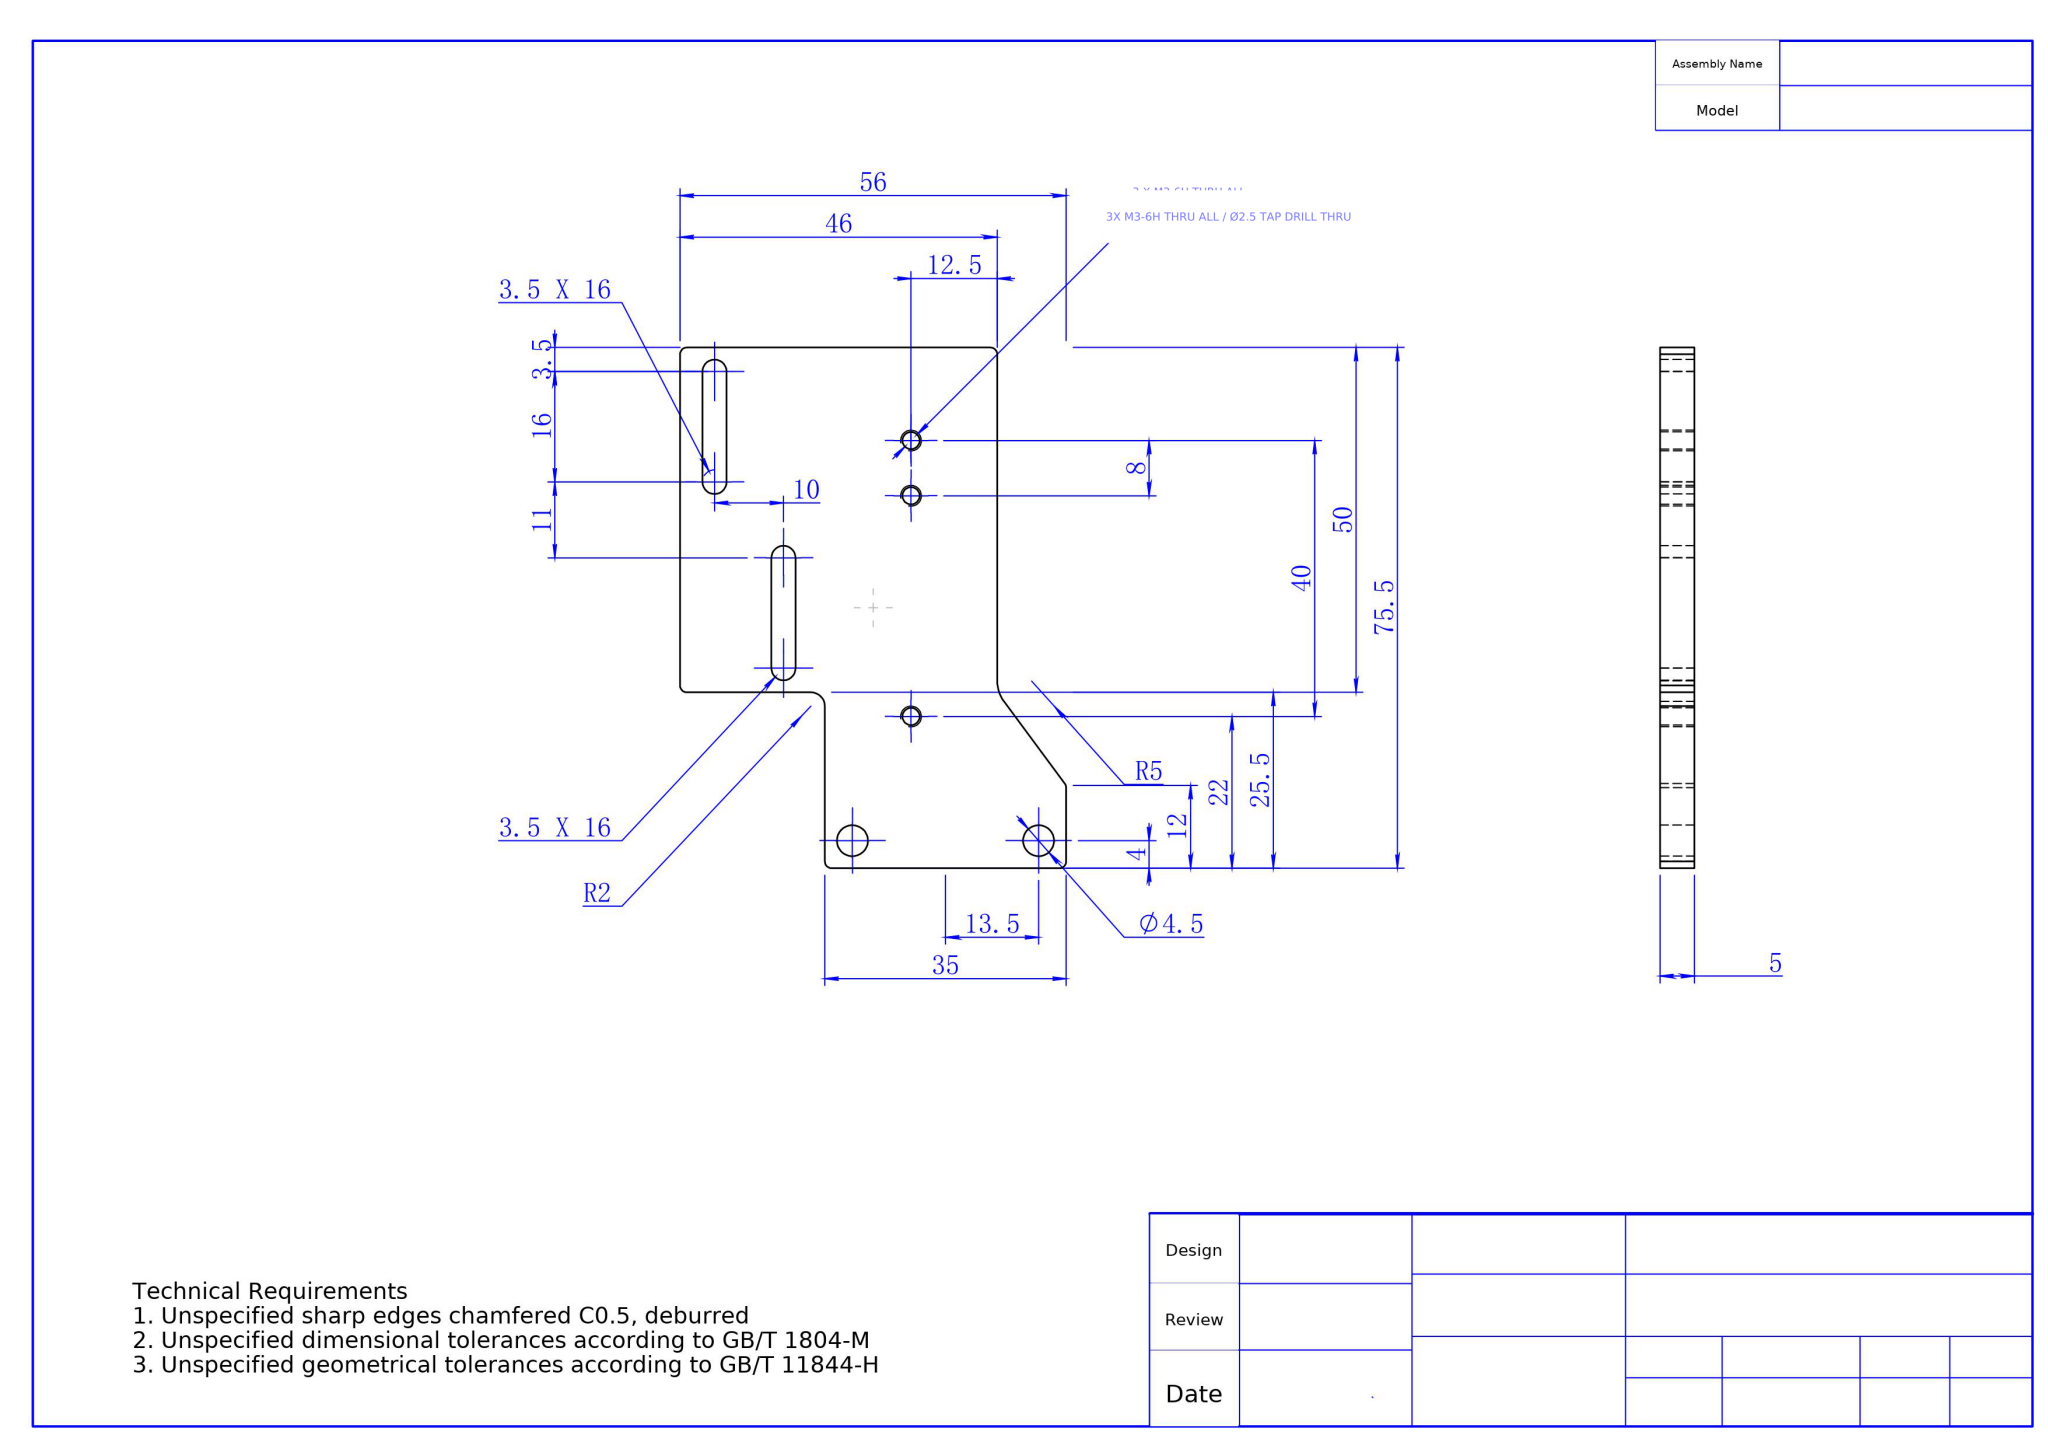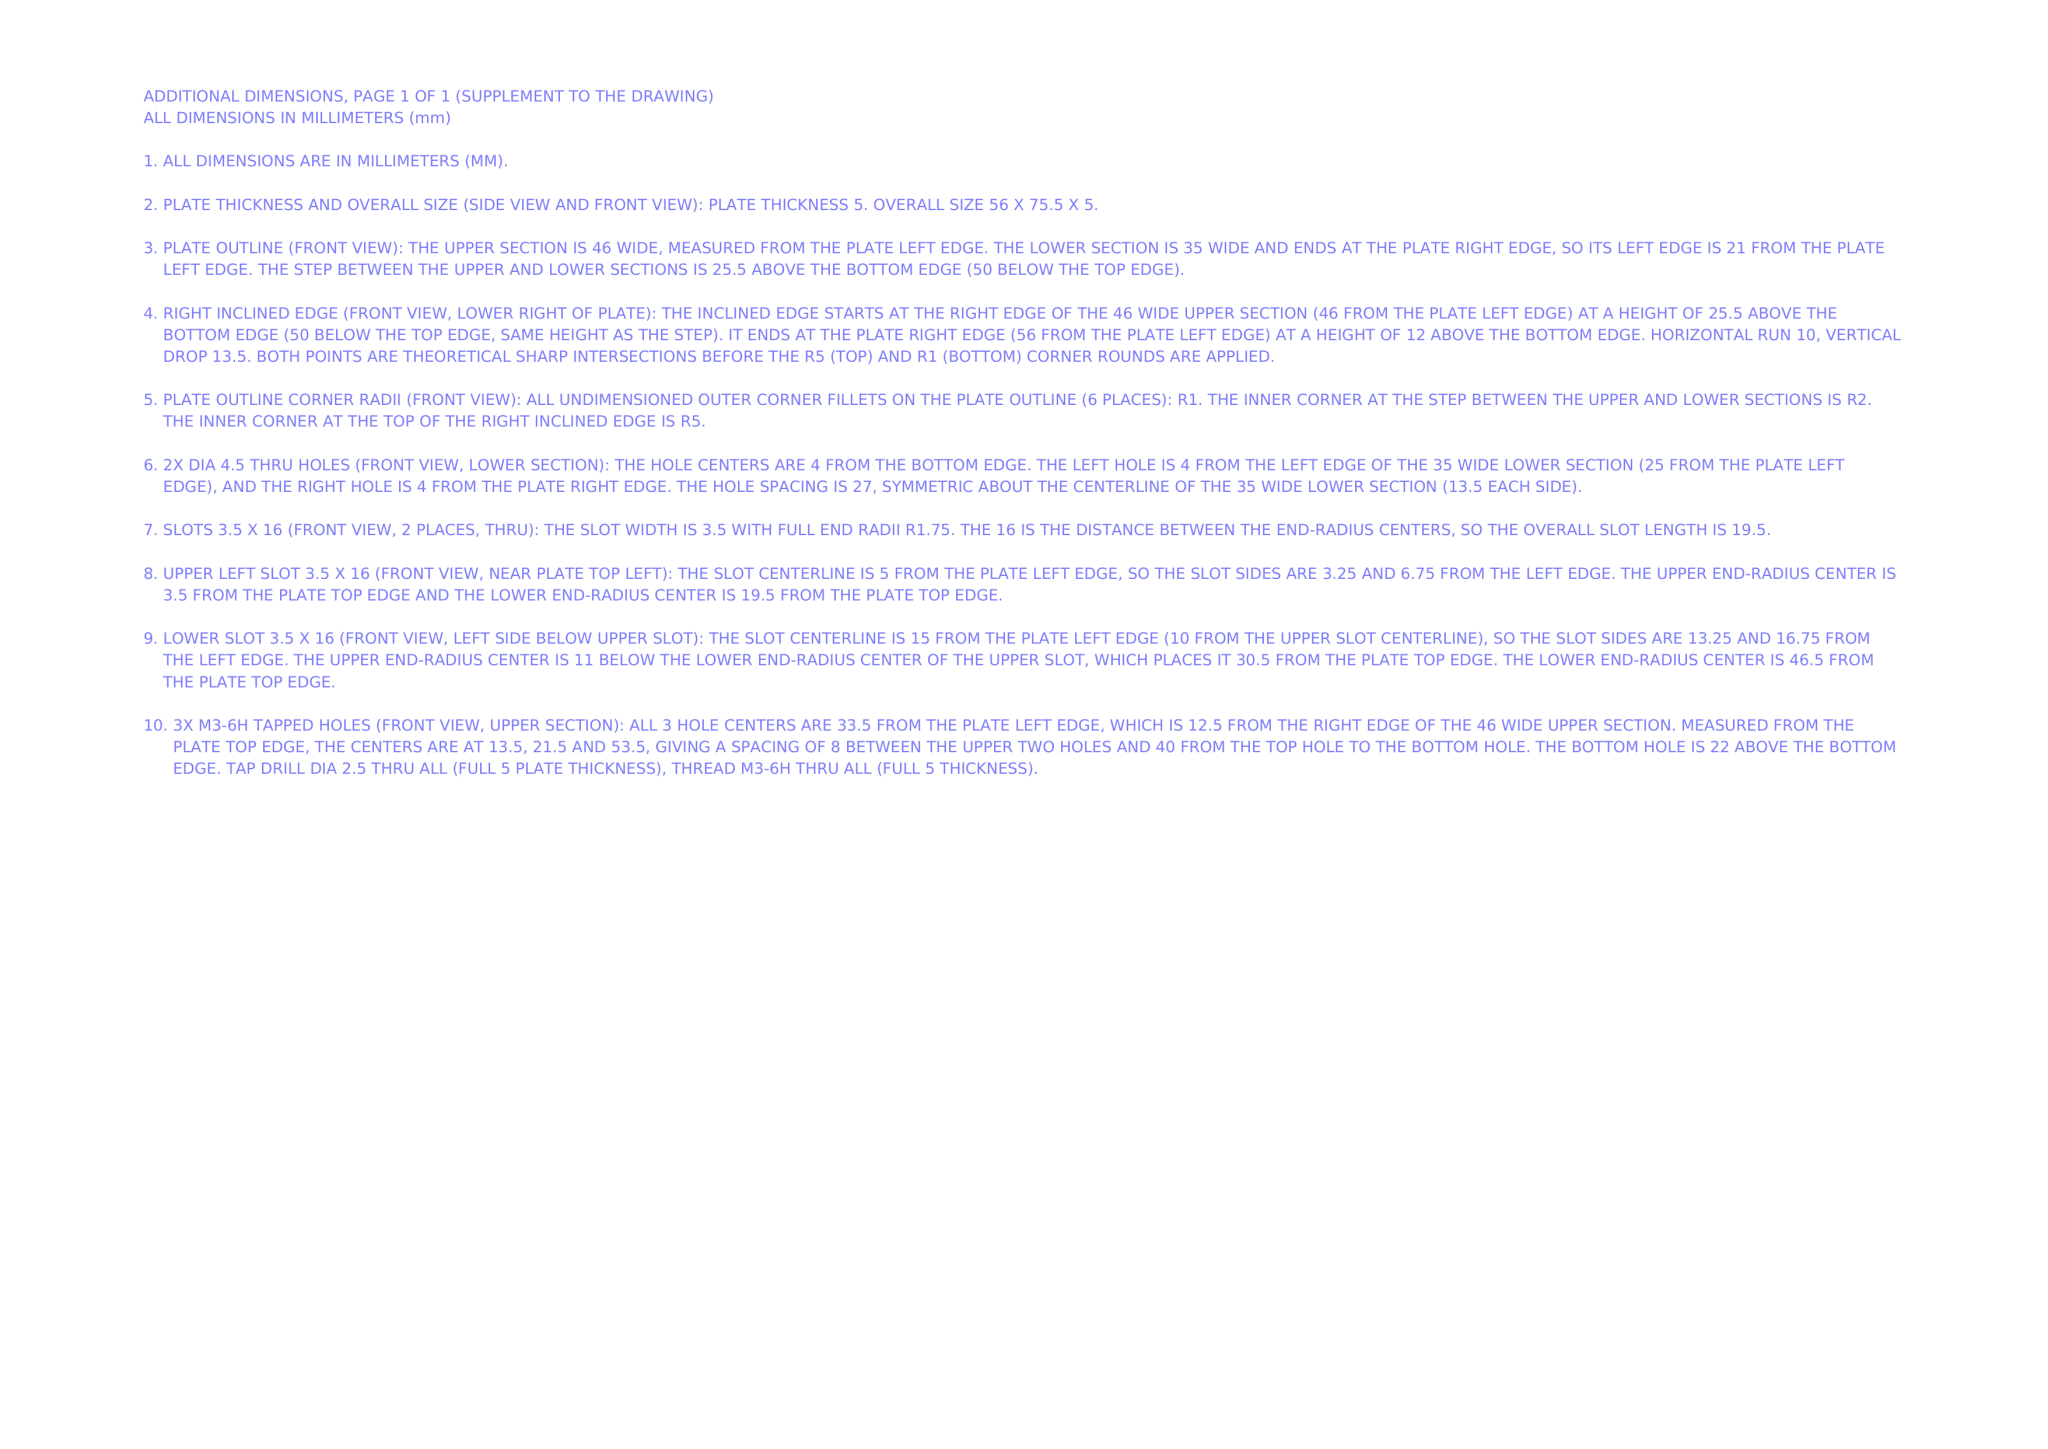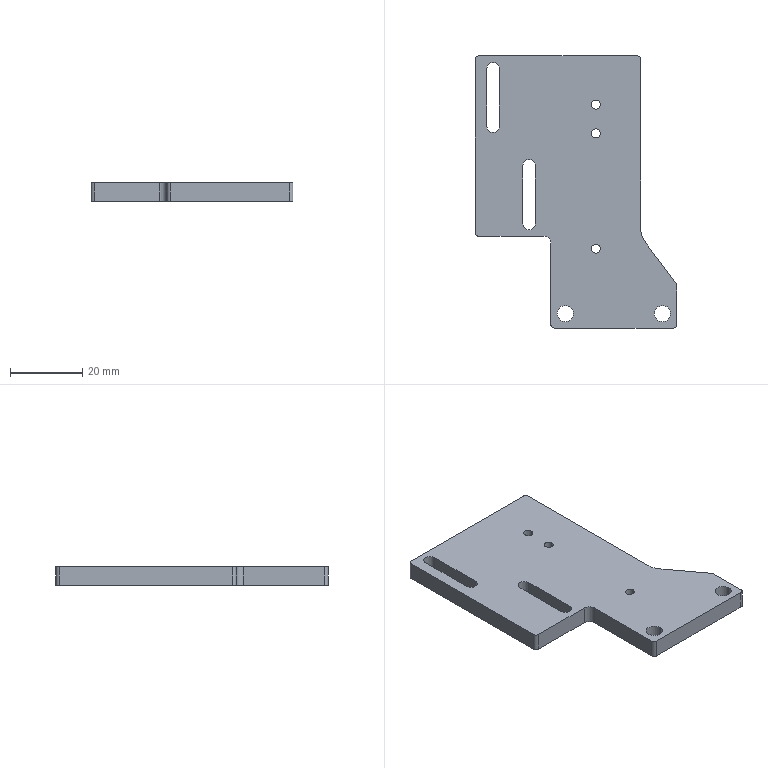Part | NX | mm | 1 solid | 36 faces | box 56 x 75.5 x 5 mm | volume 14736 mm3 | cylinder 22 | plane 14 | commonest cylinder face diameters 2.5 x6 2 x6 4.5 x4 3.5 x4 4 x1 10 x1